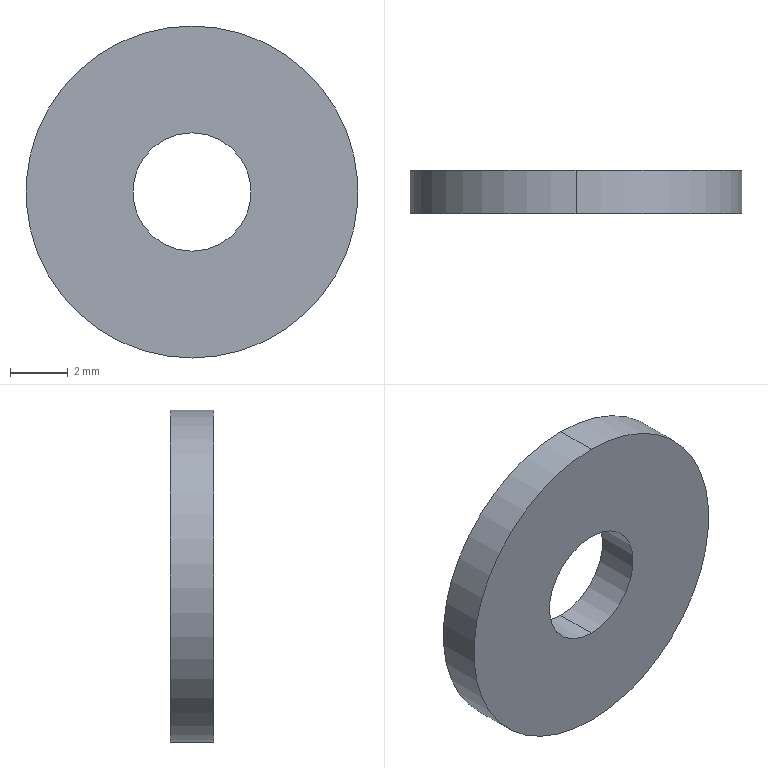Component | SolidWorks | H2020022-0408-1-11 | 1 solid | 6 faces | box 11.5 x 1.5 x 11.5 mm | volume 136 mm3 | cylinder 4 | plane 2 | commonest cylinder face diameters 4.1 x2 11.5 x2 | material Stainless Steel304
build123d program:
from build123d import *

# Parameters (mm, degrees)
SKETCH1_R           = 5.75
SKETCH1_R_2         = 2.05
BOSS_EXTRUDE1_DEPTH = 1.5


with BuildPart() as part:
    # Sketch1 → Boss-Extrude1 (new body)
    with BuildSketch(Plane(origin=(0, 0, 0), x_dir=(1, 0, 0), z_dir=(0, 1, 0))):
        with Locations(Location((0, 0, 0), (0, 0, 270))):
            Circle(SKETCH1_R)
        with Locations(Location((0, 0, 0), (0, 0, 270))):
            Circle(SKETCH1_R_2, mode=Mode.SUBTRACT)
    extrude(amount=BOSS_EXTRUDE1_DEPTH)


solid = part.part

# Placed as in the assembly
solid = solid.moved(Location((-30.964, 171.813, 280.197), (0, 0, 0)))
STEP:
#1=CARTESIAN_POINT('',(-1.219,6.823,10.951));
#2=VERTEX_POINT('',#1);
#3=CARTESIAN_POINT('',(-1.219,6.823,11.112));
#4=VERTEX_POINT('',#3);
#5=CARTESIAN_POINT('',(-1.219,6.823,11.031));
#6=DIRECTION('',(0.,1.,0.));
#7=DIRECTION('',(0.,0.,1.));
#8=AXIS2_PLACEMENT_3D('',#5,#6,#7);
#9=CIRCLE('',#8,0.08071);
#10=EDGE_CURVE('',#2,#4,#9,.T.);
#11=ORIENTED_EDGE('',*,*,#10,.T.);
#12=CARTESIAN_POINT('',(-1.219,6.764,11.112));
#13=VERTEX_POINT('',#12);
#14=CARTESIAN_POINT('',(-1.219,6.823,11.112));
#15=DIRECTION('',(0.,-1.,0.));
#16=VECTOR('',#15,39.37);
#17=LINE('',#14,#16);
#18=EDGE_CURVE('',#4,#13,#17,.T.);
#19=ORIENTED_EDGE('',*,*,#18,.T.);
#20=CARTESIAN_POINT('',(-1.219,6.764,10.951));
#21=VERTEX_POINT('',#20);
#22=CARTESIAN_POINT('',(-1.219,6.764,11.031));
#23=DIRECTION('',(0.,1.,0.));
#24=DIRECTION('',(0.,0.,1.));
#25=AXIS2_PLACEMENT_3D('',#22,#23,#24);
#26=CIRCLE('',#25,0.08071);
#27=EDGE_CURVE('',#21,#13,#26,.T.);
#28=ORIENTED_EDGE('',*,*,#27,.F.);
#29=CARTESIAN_POINT('',(-1.219,6.823,10.951));
#30=DIRECTION('',(0.,-1.,0.));
#31=VECTOR('',#30,39.37);
#32=LINE('',#29,#31);
#33=EDGE_CURVE('',#2,#21,#32,.T.);
#34=ORIENTED_EDGE('',*,*,#33,.F.);
#35=EDGE_LOOP('',(#11,#19,#28,#34));
#36=FACE_OUTER_BOUND('',#35,.T.);
#37=CARTESIAN_POINT('',(-1.219,6.823,11.031));
#38=DIRECTION('',(0.,-1.,0.));
#39=DIRECTION('',(0.,0.,-1.));
#40=AXIS2_PLACEMENT_3D('',#37,#38,#39);
#41=CYLINDRICAL_SURFACE('',#40,0.08071);
#42=ADVANCED_FACE('',(#36),#41,.F.);
#43=CARTESIAN_POINT('',(-1.219,6.823,11.258));
#44=VERTEX_POINT('',#43);
#45=CARTESIAN_POINT('',(-1.219,6.823,10.805));
#46=VERTEX_POINT('',#45);
#47=CARTESIAN_POINT('',(-1.219,6.823,11.031));
#48=DIRECTION('',(0.,1.,0.));
#49=DIRECTION('',(0.,0.,1.));
#50=AXIS2_PLACEMENT_3D('',#47,#48,#49);
#51=CIRCLE('',#50,0.2264);
#52=EDGE_CURVE('',#44,#46,#51,.T.);
#53=ORIENTED_EDGE('',*,*,#52,.F.);
#54=CARTESIAN_POINT('',(-1.219,6.764,11.258));
#55=VERTEX_POINT('',#54);
#56=CARTESIAN_POINT('',(-1.219,6.823,11.258));
#57=DIRECTION('',(0.,-1.,0.));
#58=VECTOR('',#57,39.37);
#59=LINE('',#56,#58);
#60=EDGE_CURVE('',#44,#55,#59,.T.);
#61=ORIENTED_EDGE('',*,*,#60,.T.);
#62=CARTESIAN_POINT('',(-1.219,6.764,10.805));
#63=VERTEX_POINT('',#62);
#64=CARTESIAN_POINT('',(-1.219,6.764,11.031));
#65=DIRECTION('',(0.,1.,0.));
#66=DIRECTION('',(0.,0.,1.));
#67=AXIS2_PLACEMENT_3D('',#64,#65,#66);
#68=CIRCLE('',#67,0.2264);
#69=EDGE_CURVE('',#55,#63,#68,.T.);
#70=ORIENTED_EDGE('',*,*,#69,.T.);
#71=CARTESIAN_POINT('',(-1.219,6.823,10.805));
#72=DIRECTION('',(0.,-1.,0.));
#73=VECTOR('',#72,39.37);
#74=LINE('',#71,#73);
#75=EDGE_CURVE('',#46,#63,#74,.T.);
#76=ORIENTED_EDGE('',*,*,#75,.F.);
#77=EDGE_LOOP('',(#53,#61,#70,#76));
#78=FACE_OUTER_BOUND('',#77,.T.);
#79=CARTESIAN_POINT('',(-1.219,6.823,11.031));
#80=DIRECTION('',(0.,-1.,0.));
#81=DIRECTION('',(0.,0.,-1.));
#82=AXIS2_PLACEMENT_3D('',#79,#80,#81);
#83=CYLINDRICAL_SURFACE('',#82,0.2264);
#84=ADVANCED_FACE('',(#78),#83,.T.);
#85=CARTESIAN_POINT('',(-1.219,6.823,11.031));
#86=DIRECTION('',(0.,1.,0.));
#87=DIRECTION('',(0.,0.,1.));
#88=AXIS2_PLACEMENT_3D('',#85,#86,#87);
#89=CIRCLE('',#88,0.2264);
#90=EDGE_CURVE('',#46,#44,#89,.T.);
#91=ORIENTED_EDGE('',*,*,#90,.T.);
#92=ORIENTED_EDGE('',*,*,#52,.T.);
#93=EDGE_LOOP('',(#91,#92));
#94=FACE_OUTER_BOUND('',#93,.T.);
#95=ORIENTED_EDGE('',*,*,#10,.F.);
#96=CARTESIAN_POINT('',(-1.219,6.823,11.031));
#97=DIRECTION('',(0.,1.,0.));
#98=DIRECTION('',(0.,0.,1.));
#99=AXIS2_PLACEMENT_3D('',#96,#97,#98);
#100=CIRCLE('',#99,0.08071);
#101=EDGE_CURVE('',#4,#2,#100,.T.);
#102=ORIENTED_EDGE('',*,*,#101,.F.);
#103=EDGE_LOOP('',(#95,#102));
#104=FACE_BOUND('',#103,.T.);
#105=CARTESIAN_POINT('',(-1.219,6.823,11.031));
#106=DIRECTION('',(0.,1.,0.));
#107=DIRECTION('',(0.,0.,1.));
#108=AXIS2_PLACEMENT_3D('',#105,#106,#107);
#109=PLANE('',#108);
#110=ADVANCED_FACE('',(#94,#104),#109,.T.);
#111=CARTESIAN_POINT('',(-1.219,6.764,11.031));
#112=DIRECTION('',(0.,1.,0.));
#113=DIRECTION('',(0.,0.,1.));
#114=AXIS2_PLACEMENT_3D('',#111,#112,#113);
#115=CIRCLE('',#114,0.2264);
#116=EDGE_CURVE('',#63,#55,#115,.T.);
#117=ORIENTED_EDGE('',*,*,#116,.F.);
#118=ORIENTED_EDGE('',*,*,#69,.F.);
#119=EDGE_LOOP('',(#117,#118));
#120=FACE_OUTER_BOUND('',#119,.T.);
#121=ORIENTED_EDGE('',*,*,#27,.T.);
#122=CARTESIAN_POINT('',(-1.219,6.764,11.031));
#123=DIRECTION('',(0.,1.,0.));
#124=DIRECTION('',(0.,0.,1.));
#125=AXIS2_PLACEMENT_3D('',#122,#123,#124);
#126=CIRCLE('',#125,0.08071);
#127=EDGE_CURVE('',#13,#21,#126,.T.);
#128=ORIENTED_EDGE('',*,*,#127,.T.);
#129=EDGE_LOOP('',(#121,#128));
#130=FACE_BOUND('',#129,.T.);
#131=CARTESIAN_POINT('',(-1.219,6.764,11.031));
#132=DIRECTION('',(0.,1.,0.));
#133=DIRECTION('',(0.,0.,1.));
#134=AXIS2_PLACEMENT_3D('',#131,#132,#133);
#135=PLANE('',#134);
#136=ADVANCED_FACE('',(#120,#130),#135,.F.);
#137=ORIENTED_EDGE('',*,*,#60,.F.);
#138=ORIENTED_EDGE('',*,*,#90,.F.);
#139=ORIENTED_EDGE('',*,*,#75,.T.);
#140=ORIENTED_EDGE('',*,*,#116,.T.);
#141=EDGE_LOOP('',(#137,#138,#139,#140));
#142=FACE_OUTER_BOUND('',#141,.T.);
#143=CARTESIAN_POINT('',(-1.219,6.823,11.031));
#144=DIRECTION('',(0.,-1.,0.));
#145=DIRECTION('',(0.,0.,-1.));
#146=AXIS2_PLACEMENT_3D('',#143,#144,#145);
#147=CYLINDRICAL_SURFACE('',#146,0.2264);
#148=ADVANCED_FACE('',(#142),#147,.T.);
#149=ORIENTED_EDGE('',*,*,#18,.F.);
#150=ORIENTED_EDGE('',*,*,#101,.T.);
#151=ORIENTED_EDGE('',*,*,#33,.T.);
#152=ORIENTED_EDGE('',*,*,#127,.F.);
#153=EDGE_LOOP('',(#149,#150,#151,#152));
#154=FACE_OUTER_BOUND('',#153,.T.);
#155=CARTESIAN_POINT('',(-1.219,6.823,11.031));
#156=DIRECTION('',(0.,-1.,0.));
#157=DIRECTION('',(0.,0.,-1.));
#158=AXIS2_PLACEMENT_3D('',#155,#156,#157);
#159=CYLINDRICAL_SURFACE('',#158,0.08071);
#160=ADVANCED_FACE('',(#154),#159,.F.);
#161=CLOSED_SHELL('',(#42,#84,#110,#136,#148,#160));
#162=MANIFOLD_SOLID_BREP('',#161);
#163=CARTESIAN_POINT('',(0.,0.,0.));
#164=DIRECTION('',(0.,0.,1.));
#165=DIRECTION('',(1.,0.,0.));
#166=AXIS2_PLACEMENT_3D('',#163,#164,#165);
#167=(LENGTH_UNIT()NAMED_UNIT(*)SI_UNIT($,.METRE.));
#168=LENGTH_MEASURE_WITH_UNIT(LENGTH_MEASURE(0.0254),#167);
#169=DIMENSIONAL_EXPONENTS(1.,0.,0.,0.,0.,0.,0.);
#170=(CONVERSION_BASED_UNIT('',#168)LENGTH_UNIT()NAMED_UNIT(#169));
#171=UNCERTAINTY_MEASURE_WITH_UNIT(LENGTH_MEASURE(0.00001),#170,'','');
#172=(NAMED_UNIT(*)PLANE_ANGLE_UNIT()SI_UNIT($,.RADIAN.));
#173=(NAMED_UNIT(*)SI_UNIT($,.STERADIAN.)SOLID_ANGLE_UNIT());
#174=(GEOMETRIC_REPRESENTATION_CONTEXT(3)GLOBAL_UNCERTAINTY_ASSIGNED_CONTEXT((#171))GLOBAL_UNIT_ASSIGNED_CONTEXT((#170,#172,#173))REPRESENTATION_CONTEXT('',''));
#175=ADVANCED_BREP_SHAPE_REPRESENTATION('',(#162,#166),#174);
#176=COLOUR_RGB('',0.7922,0.8196,0.9333);
#177=FILL_AREA_STYLE_COLOUR('',#176);
#178=FILL_AREA_STYLE('',(#177));
#179=SURFACE_STYLE_FILL_AREA(#178);
#180=SURFACE_SIDE_STYLE('',(#179));
#181=SURFACE_STYLE_USAGE(.BOTH.,#180);
#182=PRESENTATION_STYLE_ASSIGNMENT((#181));
#183=STYLED_ITEM('',(#182),#162);
#184=PRESENTATION_LAYER_ASSIGNMENT('','',(#183));
#185=(LENGTH_UNIT()NAMED_UNIT(*)SI_UNIT($,.METRE.));
#186=LENGTH_MEASURE_WITH_UNIT(LENGTH_MEASURE(0.0254),#185);
#187=DIMENSIONAL_EXPONENTS(1.,0.,0.,0.,0.,0.,0.);
#188=(CONVERSION_BASED_UNIT('',#186)LENGTH_UNIT()NAMED_UNIT(#187));
#189=UNCERTAINTY_MEASURE_WITH_UNIT(LENGTH_MEASURE(0.00001),#188,'','');
#190=(NAMED_UNIT(*)PLANE_ANGLE_UNIT()SI_UNIT($,.RADIAN.));
#191=(NAMED_UNIT(*)SI_UNIT($,.STERADIAN.)SOLID_ANGLE_UNIT());
#192=(GEOMETRIC_REPRESENTATION_CONTEXT(3)GLOBAL_UNCERTAINTY_ASSIGNED_CONTEXT((#189))GLOBAL_UNIT_ASSIGNED_CONTEXT((#188,#190,#191))REPRESENTATION_CONTEXT('',''));
#193=MECHANICAL_DESIGN_GEOMETRIC_PRESENTATION_REPRESENTATION('',(#183),#192);